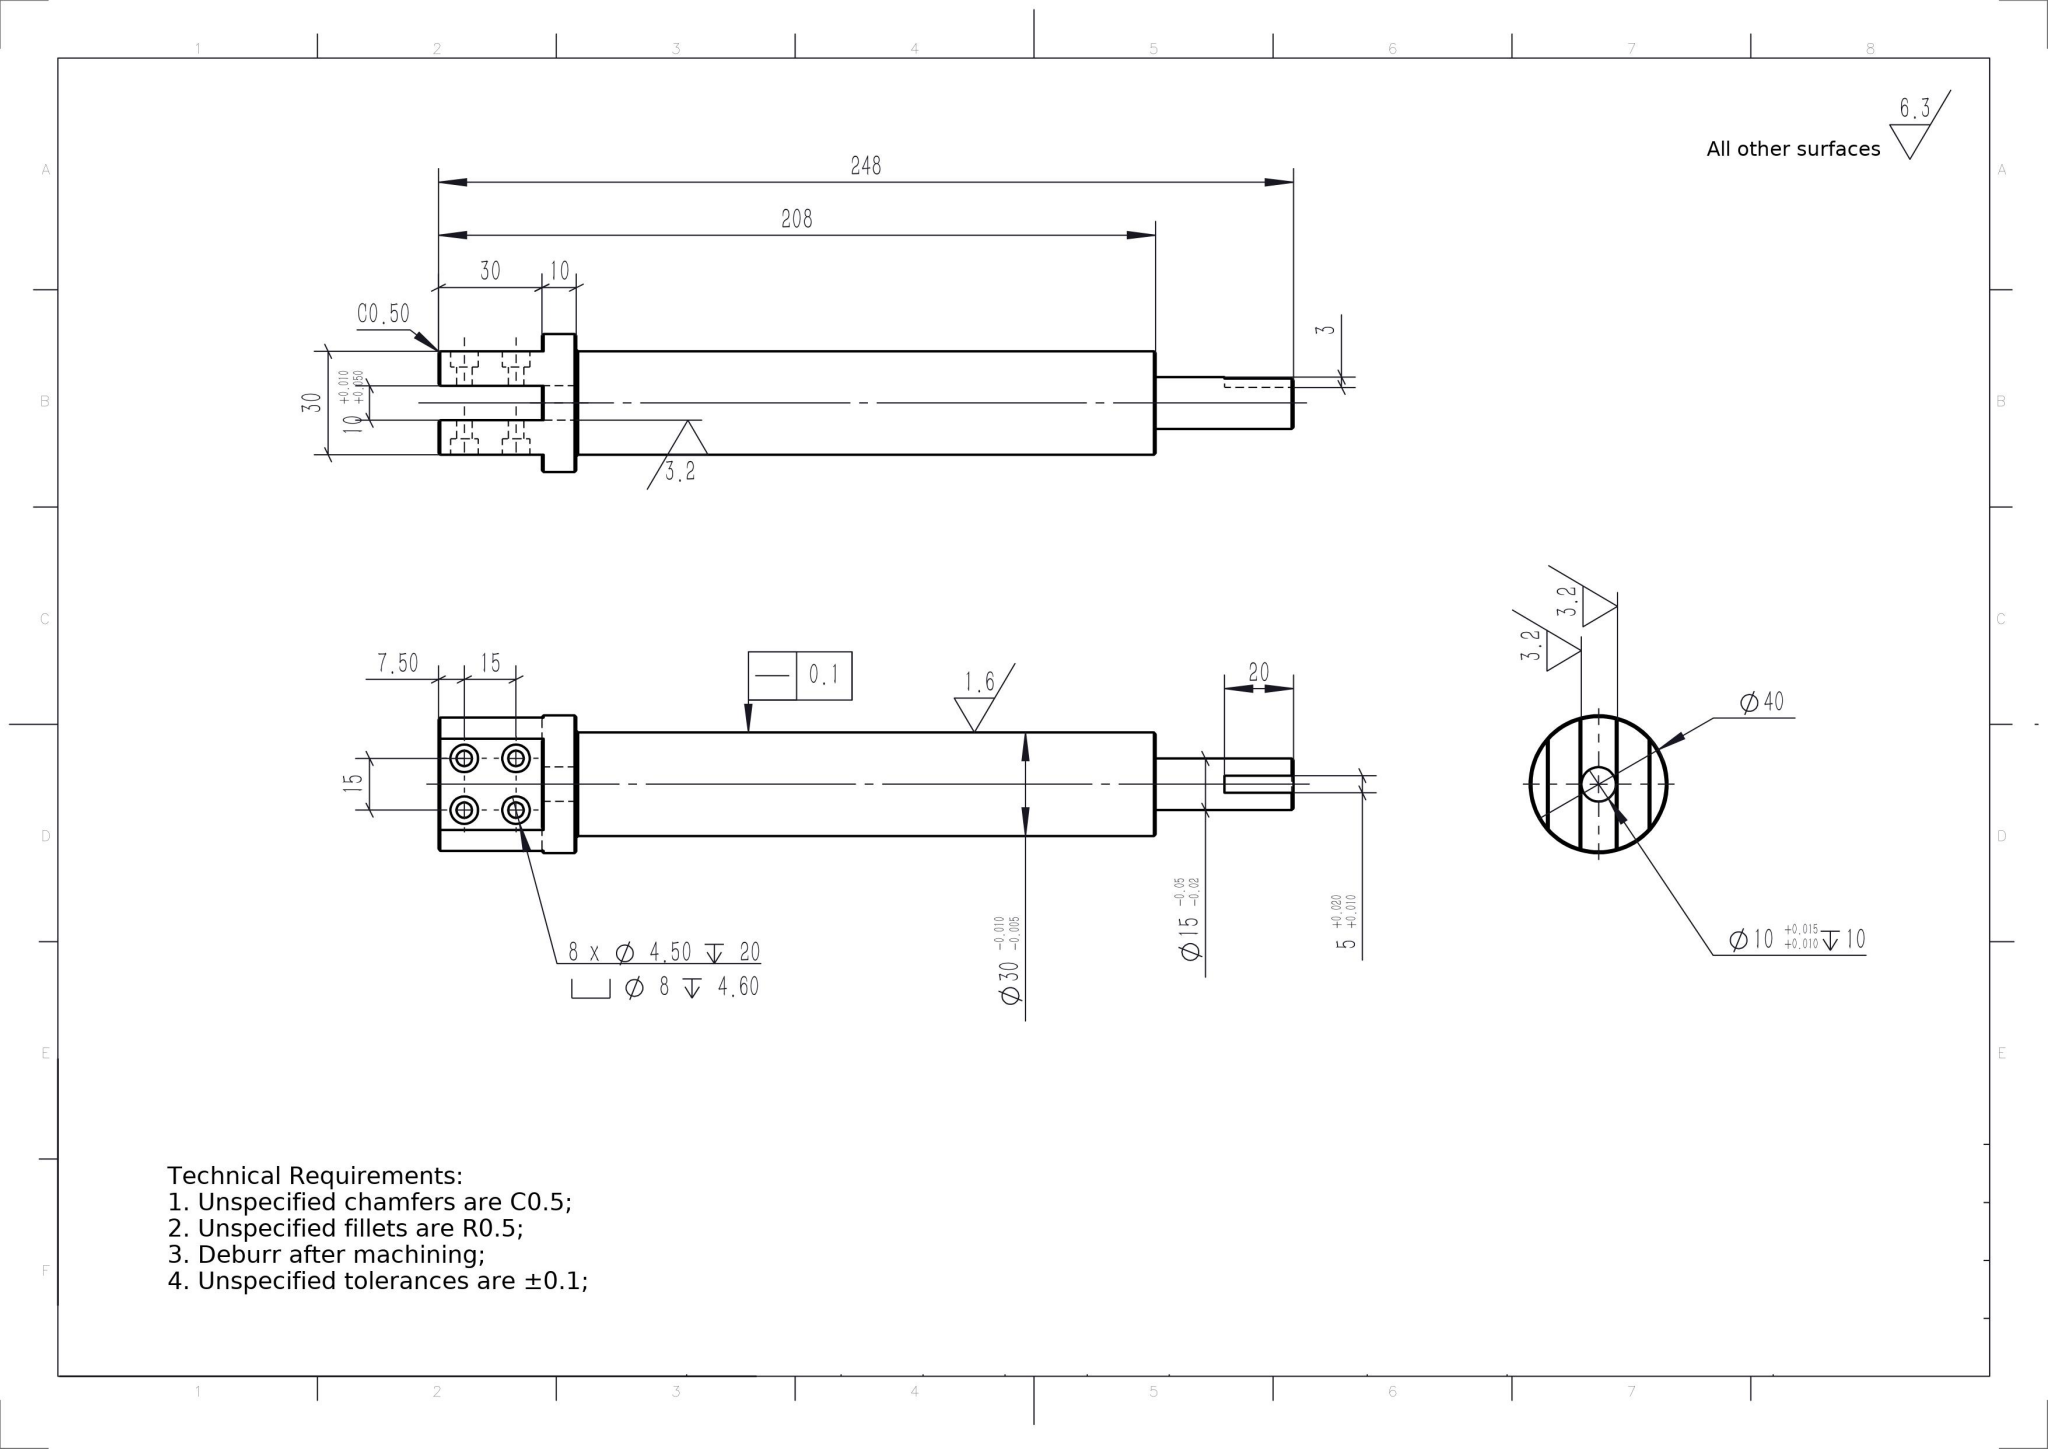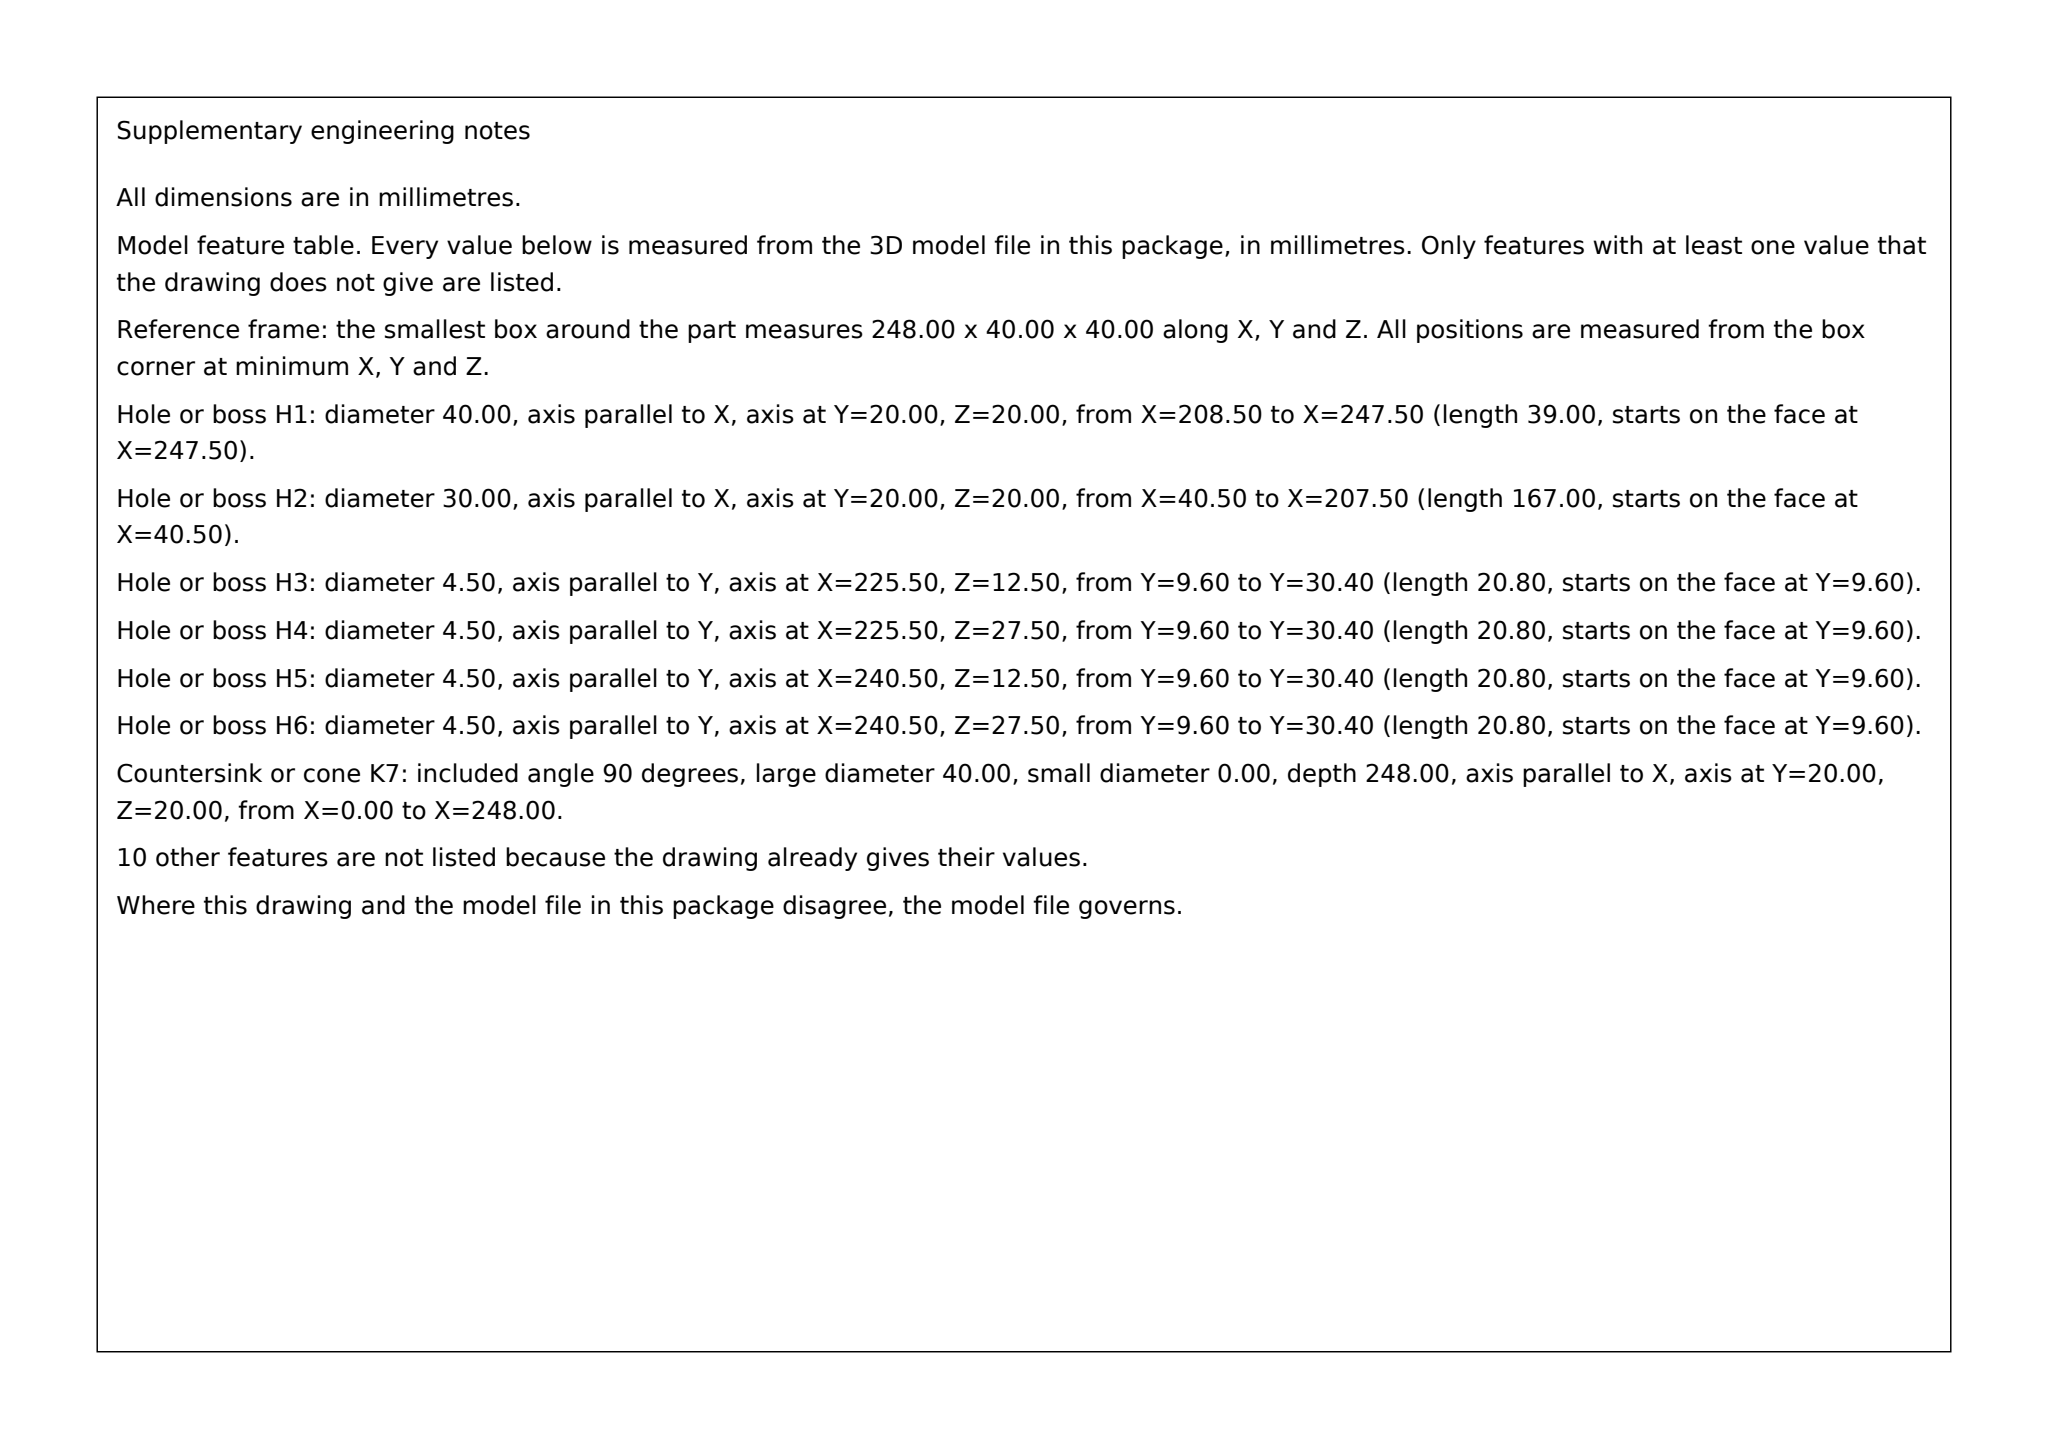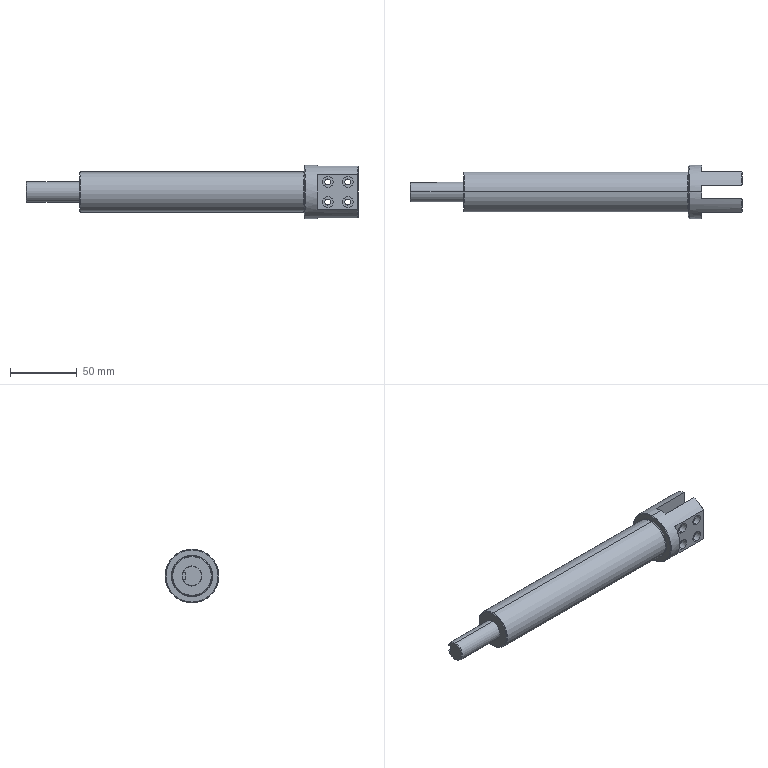Part | SolidWorks | mm | 1 solid | 88 faces | box 248 x 40 x 40 mm | volume 155113 mm3 | cylinder 40 | plane 30 | cone 18 | commonest cylinder face diameters 8 x16 4.5 x16 10 x2 40 x2 15 x2 30 x2
build123d program:
from build123d import *

# Parameters (mm, degrees)
SKETCH1_R                                         = 44
BOSS_EXTRUDE1_DEPTH                               = 400
SKETCH2_R                                         = 43
CUT_EXTRUDE1_DEPTH                                = 346
SKETCH3_R                                         = 44
BOSS_EXTRUDE2_DEPTH                               = 50
BOSS_EXTRUDE2_DRAFT                               = -30
SKETCH4_R                                         = 15
BOSS_EXTRUDE3_DEPTH                               = 170
SKETCH5_R                                         = 7.5
BOSS_EXTRUDE4_DEPTH                               = 40
CHAMFER1_SIZE                                     = 0.5
SKETCH6_W                                         = 5
SKETCH6_H                                         = 5
CUT_EXTRUDE2_DEPTH                                = 20
SKETCH7_R                                         = 50
CUT_EXTRUDE3_DEPTH                                = 452
SKETCH8_R                                         = 20
BOSS_EXTRUDE5_DEPTH                               = 40
CUT_EXTRUDE4_DEPTH                                = 30
SKETCH10_R                                        = 5
CUT_EXTRUDE5_DEPTH                                = 10
HOLE_SIZE_ACCORDING_TO_TYPE_OF_HEXAGO_D           = 4.5
HOLE_SIZE_ACCORDING_TO_TYPE_OF_HEXAGO_DEPTH       = 19.999
HOLE_SIZE_ACCORDING_TO_TYPE_OF_HEXAGO_CBORE_D     = 8
HOLE_SIZE_ACCORDING_TO_TYPE_OF_HEXAGO_CBORE_DEPTH = 4.6
CHAMFER2_SIZE                                     = 0.5


with BuildPart() as part:
    # Sketch1 → Boss-Extrude1 (new body)
    with BuildSketch(Plane(origin=(0, 0, 0), x_dir=(0, 0, -1), z_dir=(1, 0, 0))):
        Circle(SKETCH1_R)
    extrude(amount=BOSS_EXTRUDE1_DEPTH)

    # Sketch2 → Cut-Extrude1 (cut)
    with BuildSketch(Plane(origin=(0, 0, 0), x_dir=(0, 0, -1), z_dir=(1, 0, 0))):
        Circle(SKETCH2_R)
    extrude(amount=CUT_EXTRUDE1_DEPTH, mode=Mode.SUBTRACT)


with BuildPart() as boss_extrude2_tool:
    # Sketch3 → Boss-Extrude2 (with draft: the straight prism first)
    with BuildSketch(Plane(origin=(0, 0, 0), x_dir=(0, 0, -1), z_dir=(1, 0, 0))):
        Circle(SKETCH3_R)
    extrude(amount=-BOSS_EXTRUDE2_DEPTH)
    # Boss-Extrude2: the draft: its side faces are tilted about the plane it starts from
    boss_extrude2_sides = [boss_extrude2_tool.faces().sort_by_distance(p)[0] for p in [
        (-25, 0, 44),
    ]]
    draft(boss_extrude2_sides, Plane(origin=(0, 0, 0), x_dir=(0, 0, -1), z_dir=(1, 0, 0)), BOSS_EXTRUDE2_DRAFT)


with BuildPart() as part_1:
    add(part.part)

    # Boss-Extrude2: add boss_extrude2_tool
    add(boss_extrude2_tool.part)

    # Sketch4 → Boss-Extrude3 (add)
    with BuildSketch(Plane.ZY.offset(50)):
        Circle(SKETCH4_R)
    extrude(amount=BOSS_EXTRUDE3_DEPTH)

    # Sketch5 → Boss-Extrude4 (add)
    with BuildSketch(Plane.ZY.offset(220)):
        Circle(SKETCH5_R)
    extrude(amount=BOSS_EXTRUDE4_DEPTH)

    # Chamfer1
    chamfer1_edges = [part_1.edges().sort_by_distance(p)[0] for p in [
        (-220, 0, -15),
        (-260, 0, -7.5),
        (400, 0, 44),
    ]]
    chamfer(chamfer1_edges, length=CHAMFER1_SIZE)

    # Sketch6 → Cut-Extrude2 (cut)
    with BuildSketch(Plane.ZY.offset(260)):
        with Locations((0, 7)):
            Rectangle(SKETCH6_W, SKETCH6_H)
    extrude(amount=-CUT_EXTRUDE2_DEPTH, mode=Mode.SUBTRACT)

    # Sketch7 → Cut-Extrude3 (cut)
    with BuildSketch(Plane(origin=(400, 0, 0), x_dir=(0, 0, -1), z_dir=(1, 0, 0))):
        Circle(SKETCH7_R)
    extrude(amount=-CUT_EXTRUDE3_DEPTH, mode=Mode.SUBTRACT)

    # Sketch8 → Boss-Extrude5 (add)
    with BuildSketch(Plane(origin=(-52, 0, 0), x_dir=(0, 0, -1), z_dir=(1, 0, 0))):
        Circle(SKETCH8_R)
    extrude(amount=BOSS_EXTRUDE5_DEPTH)

    # Sketch9 → Cut-Extrude4 (cut)
    with BuildSketch(Plane(origin=(-12, 0, 0), x_dir=(0, 0, -1), z_dir=(1, 0, 0))):
        with BuildLine():
            Line((-29.58, 5), (29.58, 5))
            ThreePointArc((29.58, 5), (30, 0), (29.58, -5))
            Line((29.58, -5), (-29.58, -5))
            ThreePointArc((-29.58, -5), (-30, 0), (-29.58, 5))
        make_face()
        with BuildLine():
            Line((-20.385, 15), (20.385, 15))
            ThreePointArc((20.385, 15), (0, 25.309), (-20.385, 15))
        make_face()
        with BuildLine():
            Line((-20.385, -15), (20.385, -15))
            ThreePointArc((20.385, -15), (0, -25.309), (-20.385, -15))
        make_face()
    extrude(amount=-CUT_EXTRUDE4_DEPTH, mode=Mode.SUBTRACT)

    # Sketch10 → Cut-Extrude5 (cut)
    with BuildSketch(Plane(origin=(-42, 0, 0), x_dir=(0, 0, -1), z_dir=(1, 0, 0))):
        Circle(SKETCH10_R)
    extrude(amount=-CUT_EXTRUDE5_DEPTH, mode=Mode.SUBTRACT)

    # Hole Size _ according to_ Type of Hexago
    with Locations(Plane(origin=(0, 15, 0), x_dir=(1, 0, 0), z_dir=(0, 1, 0))):
        with Locations((-34.5, 7.5), (-19.5, 7.5), (-19.5, -7.5), (-34.5, -7.5)):
            hole_size_according_to_type_of_hexago = CounterBoreHole(HOLE_SIZE_ACCORDING_TO_TYPE_OF_HEXAGO_D / 2, HOLE_SIZE_ACCORDING_TO_TYPE_OF_HEXAGO_CBORE_D / 2, HOLE_SIZE_ACCORDING_TO_TYPE_OF_HEXAGO_CBORE_DEPTH, depth=HOLE_SIZE_ACCORDING_TO_TYPE_OF_HEXAGO_DEPTH)

    # Mirror1: Hole Size _ according to_ Type of Hexago across plane
    add(hole_size_according_to_type_of_hexago.mirror(Plane.ZX), mode=Mode.SUBTRACT)

    # Chamfer2
    chamfer2_edges = [part_1.edges().sort_by_distance(p)[0] for p in [
        (-52, 0, -15),
        (-52, 0, 20),
        (-12, 10.46, -17.047),
        (-12, 10.46, 17.047),
        (-12, -10.46, 17.047),
        (-12, -10.46, -17.047),
        (-12, -15, 0),
        (-12, -5, 0),
        (-12, 5, 0),
        (-12, 15, 0),
        (-42, -20, 0),
        (-42, -2.52, -19.841),
        (-42, 0, 20),
        (-42, 20, 0),
    ]]
    chamfer(chamfer2_edges, length=CHAMFER2_SIZE)


solid = part_1.part